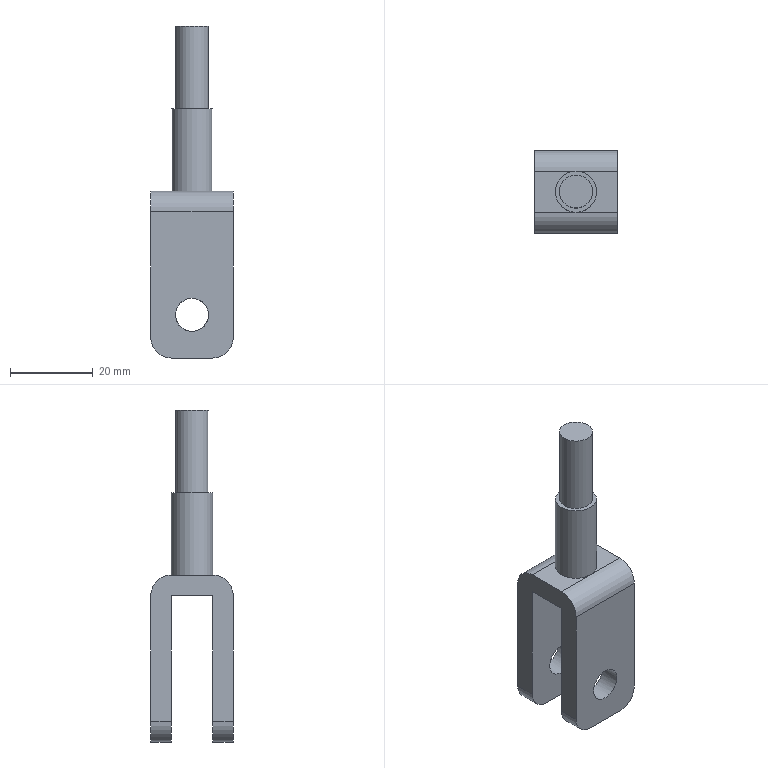Component | NX | FRONT_WHEEL_SUPPORT | 1 solid | 23 faces | volume 10840 mm3 | plane 13 | cylinder 10 | commonest cylinder face diameters 10 x7 8 x3